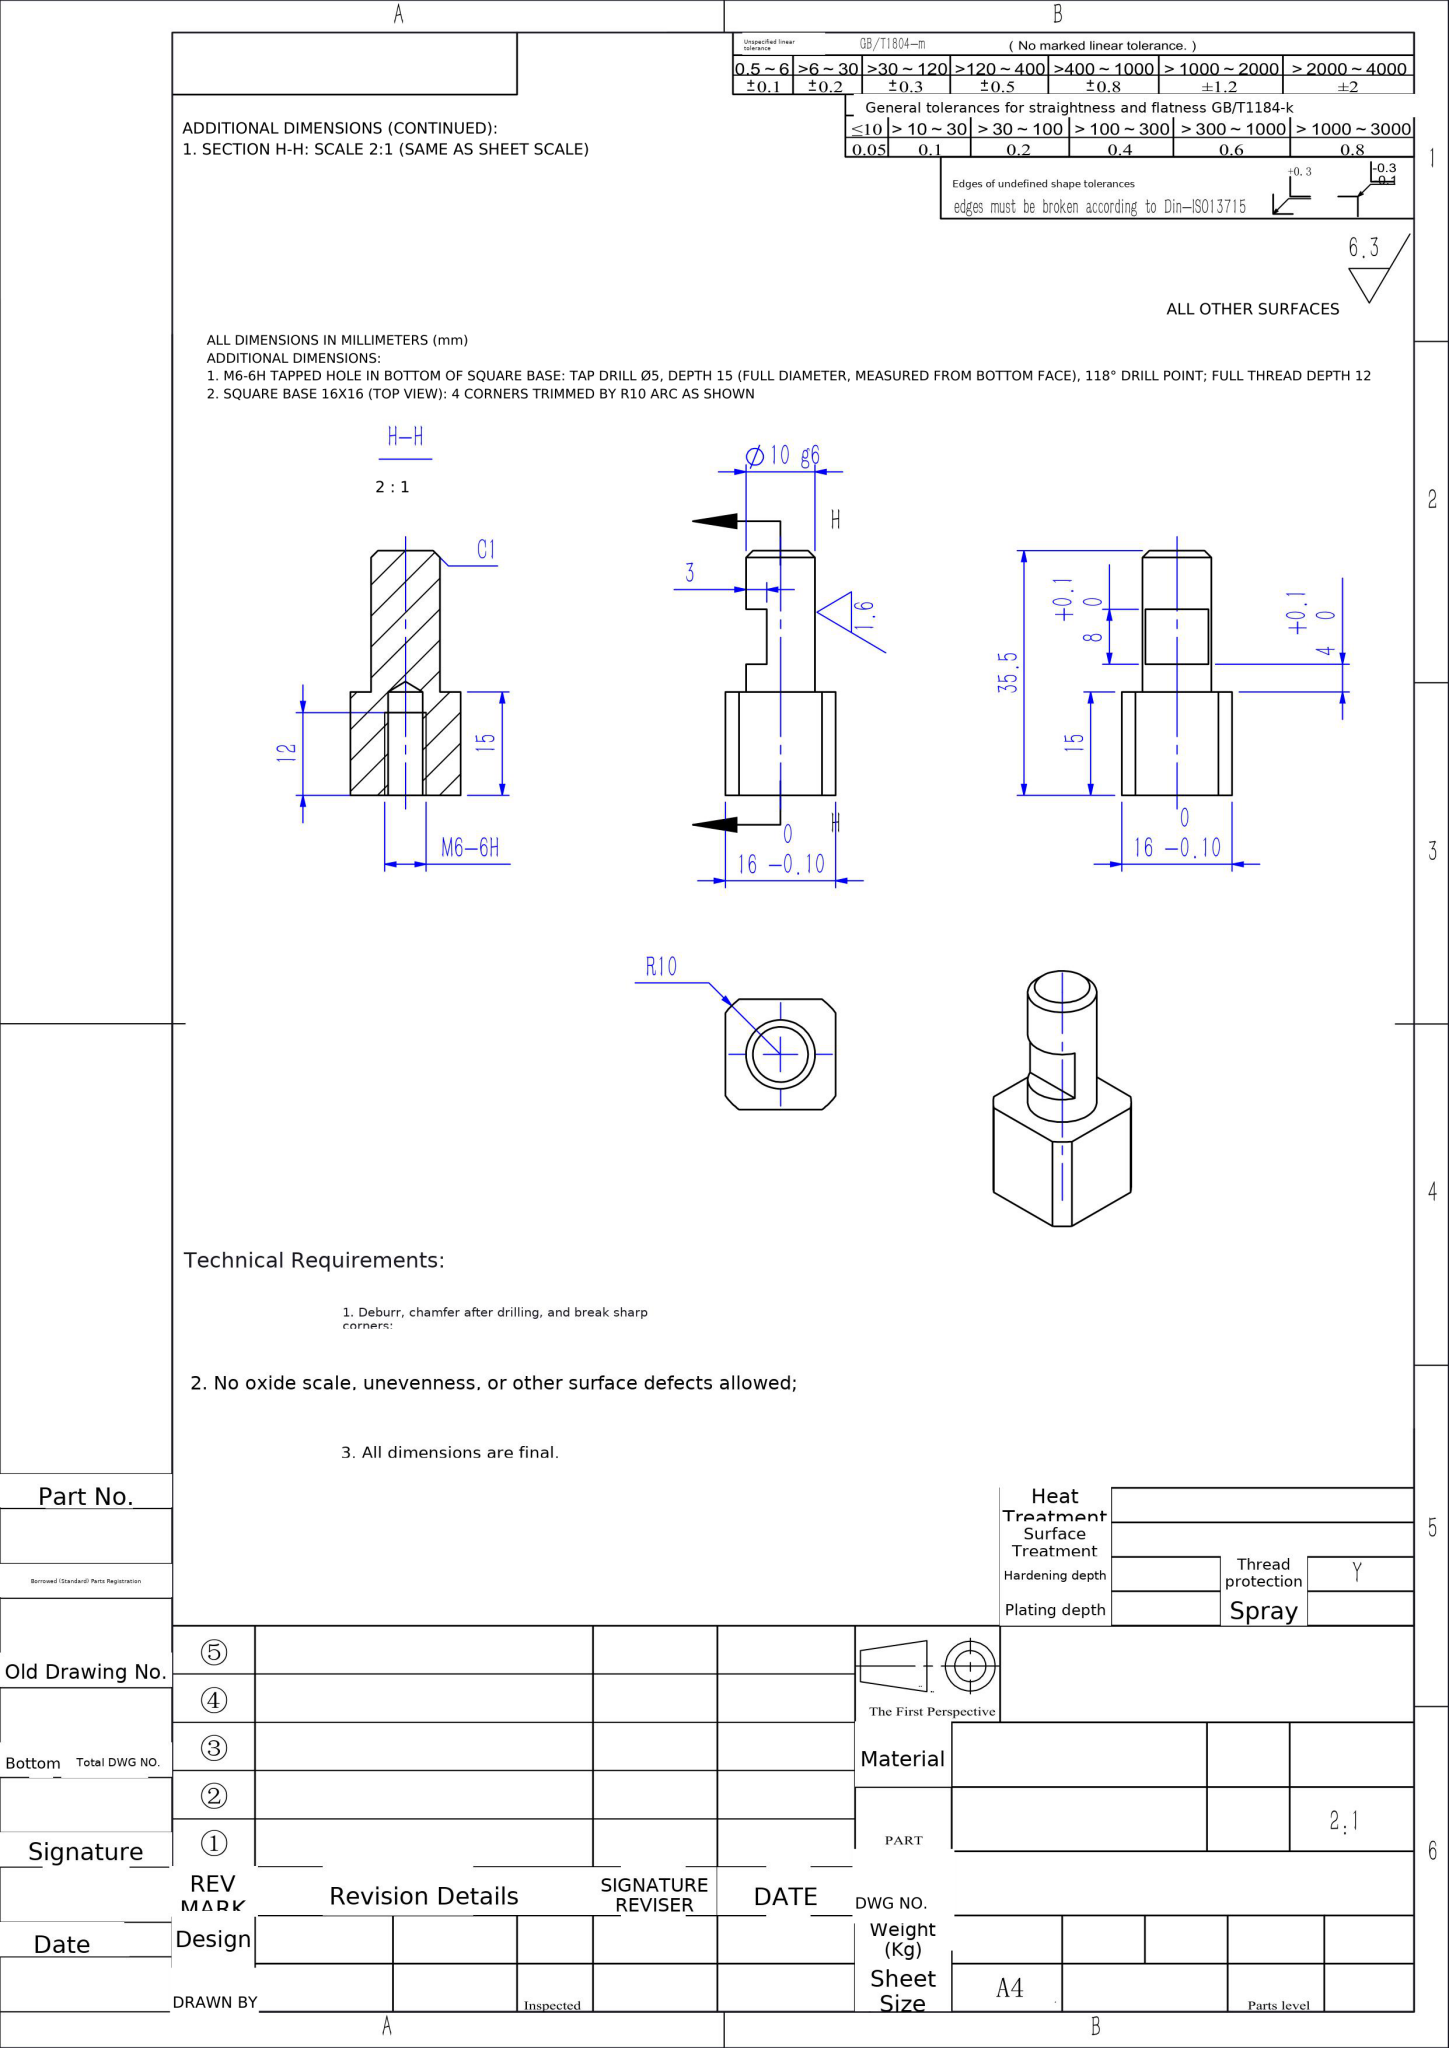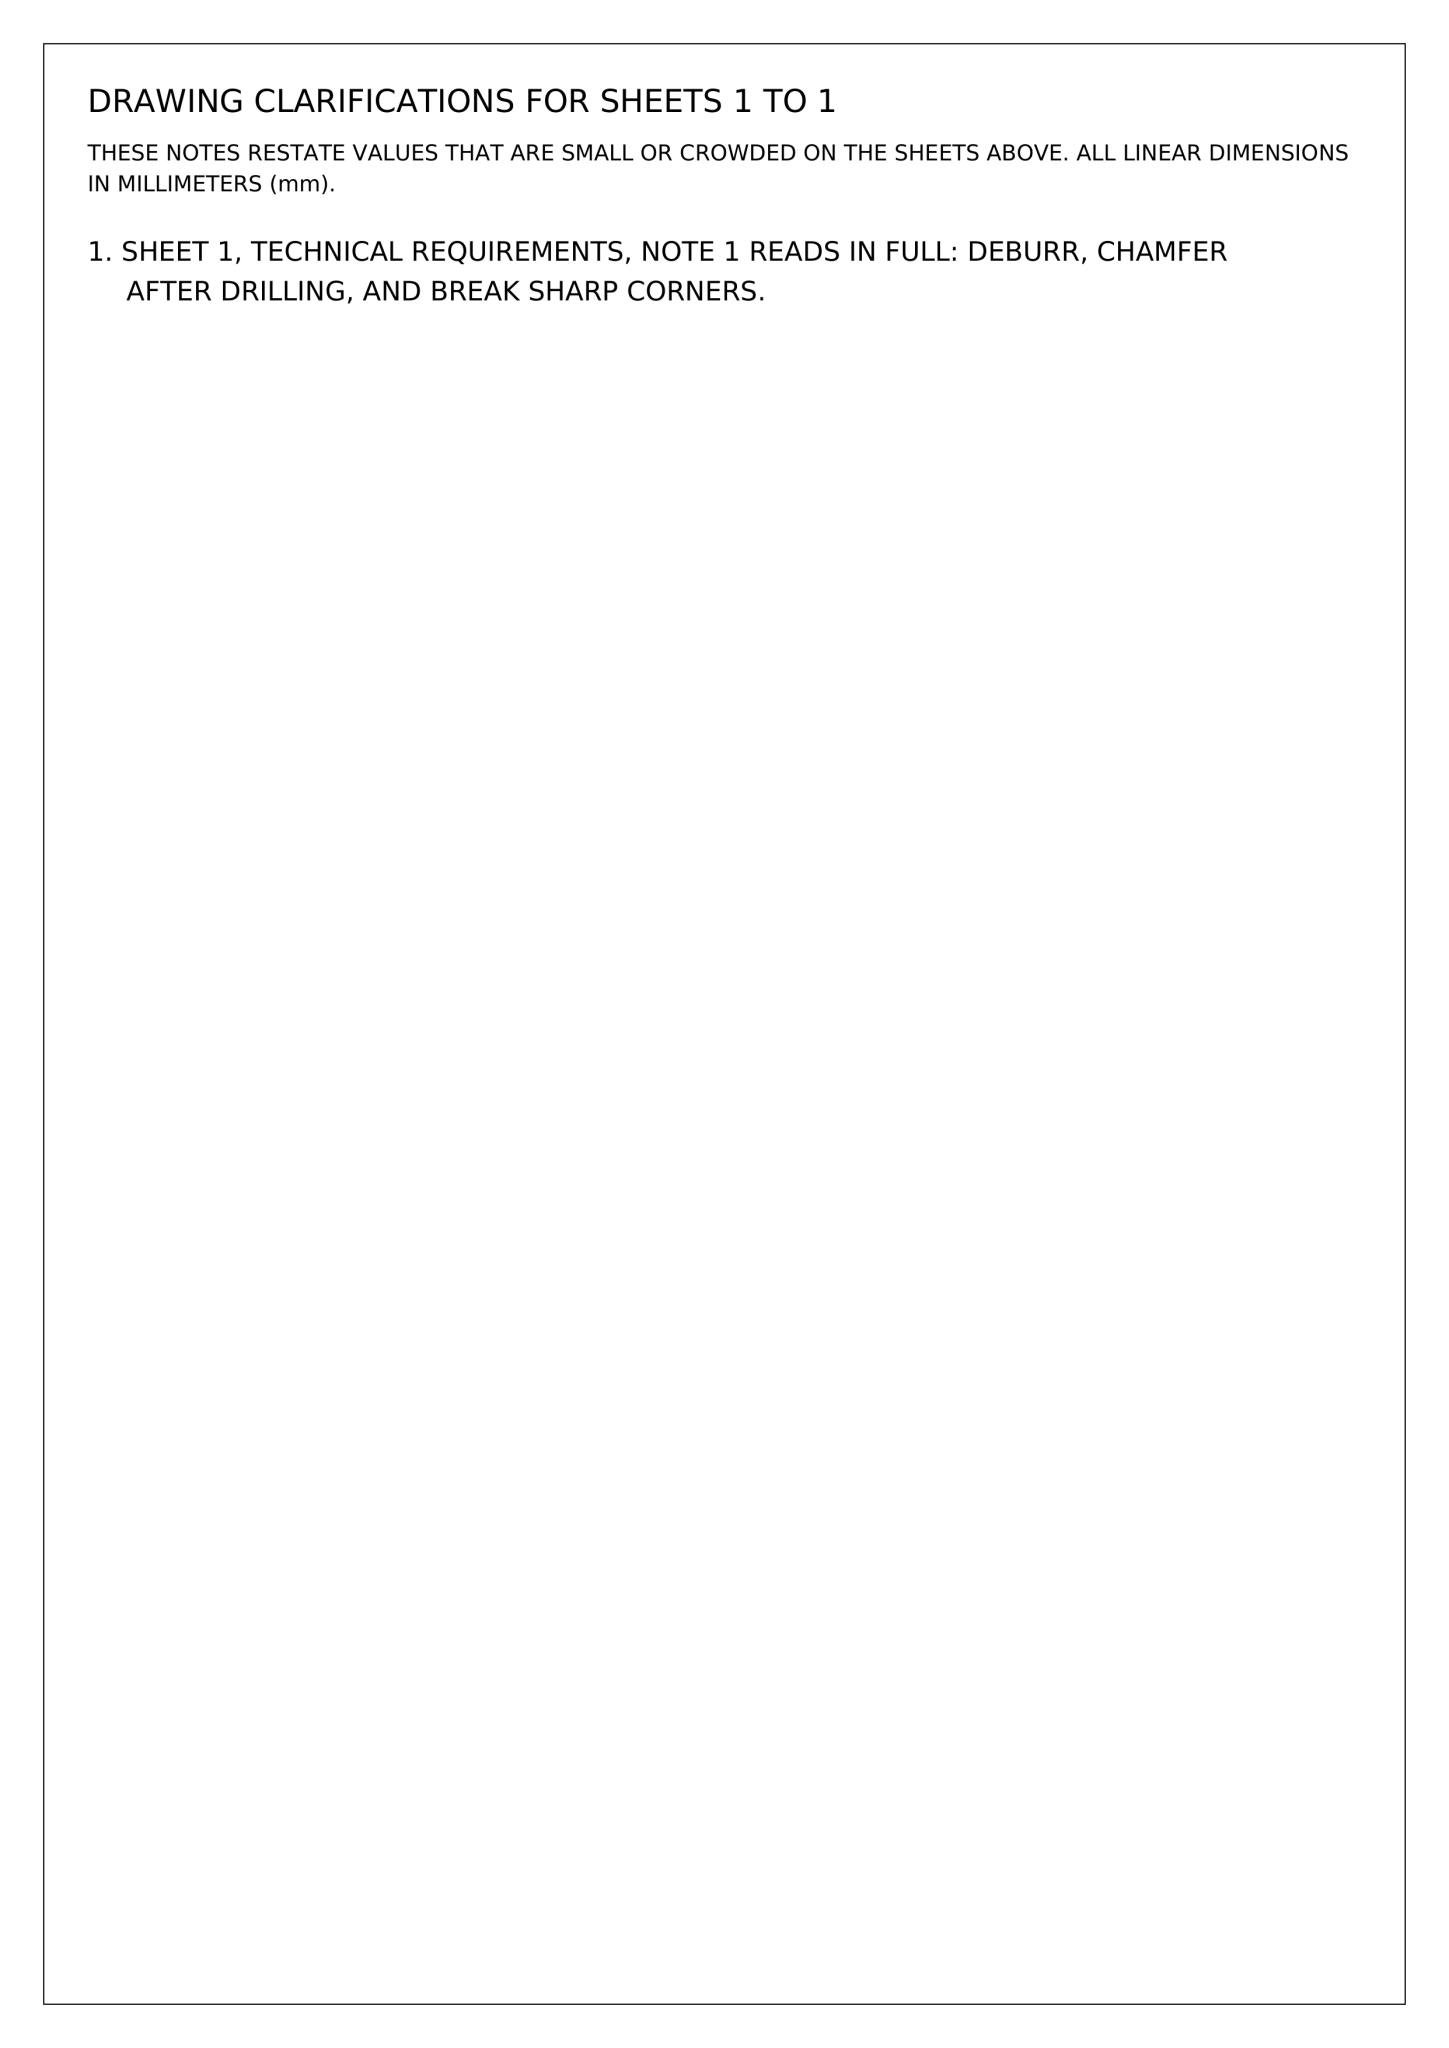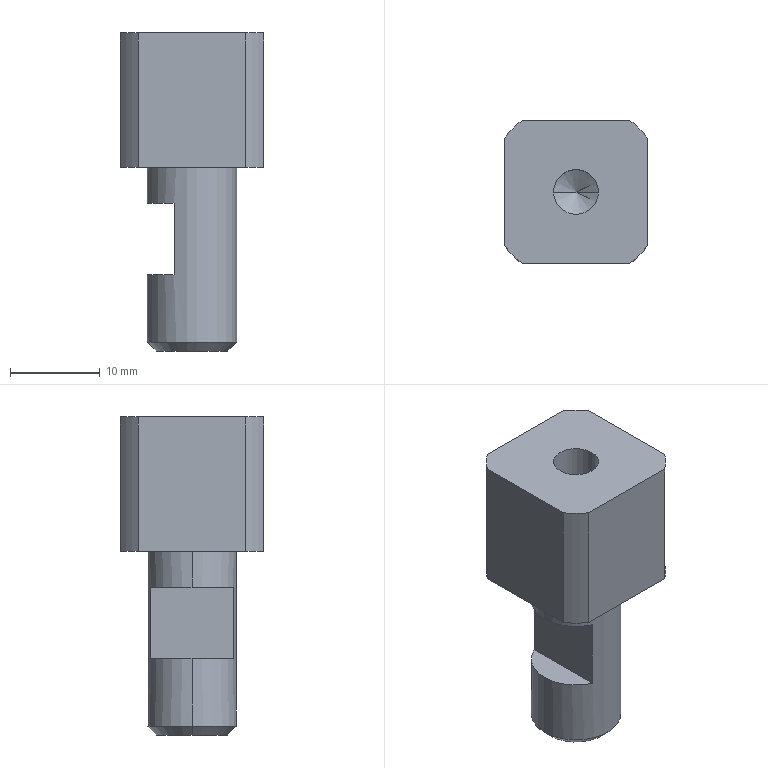Part | NX | mm | 1 solid | 22 faces | box 16 x 16 x 35.5 mm | volume 4864 mm3 | plane 10 | cylinder 8 | cone 4 | commonest cylinder face diameters 20 x4 5 x2 10 x2
STEP:
#1=COLOUR_RGB('',0.6471,0.6196,0.5882);
#2=FILL_AREA_STYLE_COLOUR('',#1);
#3=FILL_AREA_STYLE('',(#2));
#4=SURFACE_STYLE_FILL_AREA(#3);
#5=SURFACE_SIDE_STYLE('',(#4));
#6=SURFACE_STYLE_USAGE(.BOTH.,#5);
#7=PRESENTATION_STYLE_ASSIGNMENT((#6));
#8=CARTESIAN_POINT('',(-2.5,0.,20.5));
#9=VERTEX_POINT('',#8);
#10=CARTESIAN_POINT('',(2.5,0.,20.5));
#11=VERTEX_POINT('',#10);
#12=CARTESIAN_POINT('',(0.,0.,20.5));
#13=DIRECTION('',(0.,0.,1.));
#14=DIRECTION('',(1.,0.,0.));
#15=AXIS2_PLACEMENT_3D('',#12,#13,#14);
#16=CIRCLE('',#15,2.5);
#17=EDGE_CURVE('',#9,#11,#16,.T.);
#18=ORIENTED_EDGE('',*,*,#17,.F.);
#19=CARTESIAN_POINT('',(-2.5,0.,35.5));
#20=VERTEX_POINT('',#19);
#21=CARTESIAN_POINT('',(-2.5,0.,35.5));
#22=DIRECTION('',(0.,0.,1.));
#23=VECTOR('',#22,1000.);
#24=LINE('',#21,#23);
#25=EDGE_CURVE('',#9,#20,#24,.T.);
#26=ORIENTED_EDGE('',*,*,#25,.T.);
#27=CARTESIAN_POINT('',(2.5,0.,35.5));
#28=VERTEX_POINT('',#27);
#29=CARTESIAN_POINT('',(0.,0.,35.5));
#30=DIRECTION('',(0.,0.,1.));
#31=DIRECTION('',(1.,0.,0.));
#32=AXIS2_PLACEMENT_3D('',#29,#30,#31);
#33=CIRCLE('',#32,2.5);
#34=EDGE_CURVE('',#20,#28,#33,.T.);
#35=ORIENTED_EDGE('',*,*,#34,.T.);
#36=CARTESIAN_POINT('',(2.5,0.,35.5));
#37=DIRECTION('',(0.,0.,1.));
#38=VECTOR('',#37,1000.);
#39=LINE('',#36,#38);
#40=EDGE_CURVE('',#11,#28,#39,.T.);
#41=ORIENTED_EDGE('',*,*,#40,.F.);
#42=EDGE_LOOP('',(#18,#26,#35,#41));
#43=FACE_OUTER_BOUND('',#42,.T.);
#44=CARTESIAN_POINT('',(0.,0.,35.5));
#45=DIRECTION('',(0.,0.,1.));
#46=DIRECTION('',(1.,0.,0.));
#47=AXIS2_PLACEMENT_3D('',#44,#45,#46);
#48=CYLINDRICAL_SURFACE('',#47,2.5);
#49=ADVANCED_FACE('',(#43),#48,.F.);
#50=STYLED_ITEM('',(#7),#49);
#51=PRESENTATION_LAYER_ASSIGNMENT('','',(#50));
#52=(LENGTH_UNIT()NAMED_UNIT(*)SI_UNIT(.MILLI.,.METRE.));
#53=UNCERTAINTY_MEASURE_WITH_UNIT(LENGTH_MEASURE(0.00001),#52,'','');
#54=(NAMED_UNIT(*)PLANE_ANGLE_UNIT()SI_UNIT($,.RADIAN.));
#55=(NAMED_UNIT(*)SI_UNIT($,.STERADIAN.)SOLID_ANGLE_UNIT());
#56=(GEOMETRIC_REPRESENTATION_CONTEXT(3)GLOBAL_UNCERTAINTY_ASSIGNED_CONTEXT((#53))GLOBAL_UNIT_ASSIGNED_CONTEXT((#52,#54,#55))REPRESENTATION_CONTEXT('',''));
#57=MECHANICAL_DESIGN_GEOMETRIC_PRESENTATION_REPRESENTATION('',(#50),#56);
#58=COLOUR_RGB('',0.6471,0.6196,0.5882);
#59=FILL_AREA_STYLE_COLOUR('',#58);
#60=FILL_AREA_STYLE('',(#59));
#61=SURFACE_STYLE_FILL_AREA(#60);
#62=SURFACE_SIDE_STYLE('',(#61));
#63=SURFACE_STYLE_USAGE(.BOTH.,#62);
#64=PRESENTATION_STYLE_ASSIGNMENT((#63));
#65=CARTESIAN_POINT('',(-4.,0.,0.));
#66=VERTEX_POINT('',#65);
#67=CARTESIAN_POINT('',(4.,0.,0.));
#68=VERTEX_POINT('',#67);
#69=CARTESIAN_POINT('',(0.,0.,0.));
#70=DIRECTION('',(0.,0.,-1.));
#71=DIRECTION('',(1.,0.,0.));
#72=AXIS2_PLACEMENT_3D('',#69,#70,#71);
#73=CIRCLE('',#72,4.);
#74=EDGE_CURVE('',#66,#68,#73,.T.);
#75=ORIENTED_EDGE('',*,*,#74,.F.);
#76=CARTESIAN_POINT('',(-5.,0.,1.));
#77=VERTEX_POINT('',#76);
#78=CARTESIAN_POINT('',(-5.,0.,1.));
#79=DIRECTION('',(-0.7071,0.,0.7071));
#80=VECTOR('',#79,1000.);
#81=LINE('',#78,#80);
#82=EDGE_CURVE('',#66,#77,#81,.T.);
#83=ORIENTED_EDGE('',*,*,#82,.T.);
#84=CARTESIAN_POINT('',(5.,0.,1.));
#85=VERTEX_POINT('',#84);
#86=CARTESIAN_POINT('',(0.,0.,1.));
#87=DIRECTION('',(0.,0.,1.));
#88=DIRECTION('',(1.,0.,0.));
#89=AXIS2_PLACEMENT_3D('',#86,#87,#88);
#90=CIRCLE('',#89,5.);
#91=EDGE_CURVE('',#85,#77,#90,.T.);
#92=ORIENTED_EDGE('',*,*,#91,.F.);
#93=CARTESIAN_POINT('',(5.,0.,1.));
#94=DIRECTION('',(0.7071,0.,0.7071));
#95=VECTOR('',#94,1000.);
#96=LINE('',#93,#95);
#97=EDGE_CURVE('',#68,#85,#96,.T.);
#98=ORIENTED_EDGE('',*,*,#97,.F.);
#99=EDGE_LOOP('',(#75,#83,#92,#98));
#100=FACE_OUTER_BOUND('',#99,.T.);
#101=CARTESIAN_POINT('',(0.,0.,1.));
#102=DIRECTION('',(0.,0.,1.));
#103=DIRECTION('',(1.,0.,0.));
#104=AXIS2_PLACEMENT_3D('',#101,#102,#103);
#105=CONICAL_SURFACE('',#104,5.,0.7854);
#106=ADVANCED_FACE('',(#100),#105,.T.);
#107=CARTESIAN_POINT('',(-0.,0.,18.998));
#108=VERTEX_POINT('',#107);
#109=CARTESIAN_POINT('',(2.5,0.,20.5));
#110=DIRECTION('',(0.8572,0.,0.515));
#111=VECTOR('',#110,1000.);
#112=LINE('',#109,#111);
#113=EDGE_CURVE('',#108,#11,#112,.T.);
#114=ORIENTED_EDGE('',*,*,#113,.F.);
#115=CARTESIAN_POINT('',(-2.5,0.,20.5));
#116=DIRECTION('',(-0.8572,0.,0.515));
#117=VECTOR('',#116,1000.);
#118=LINE('',#115,#117);
#119=EDGE_CURVE('',#108,#9,#118,.T.);
#120=ORIENTED_EDGE('',*,*,#119,.T.);
#121=ORIENTED_EDGE('',*,*,#17,.T.);
#122=EDGE_LOOP('',(#114,#120,#121));
#123=FACE_OUTER_BOUND('',#122,.T.);
#124=CARTESIAN_POINT('',(0.,0.,20.5));
#125=DIRECTION('',(0.,0.,1.));
#126=DIRECTION('',(1.,0.,0.));
#127=AXIS2_PLACEMENT_3D('',#124,#125,#126);
#128=CONICAL_SURFACE('',#127,2.5,1.03);
#129=ADVANCED_FACE('',(#123),#128,.F.);
#130=CARTESIAN_POINT('',(5.,0.,20.5));
#131=VERTEX_POINT('',#130);
#132=CARTESIAN_POINT('',(-5.,0.,20.5));
#133=VERTEX_POINT('',#132);
#134=CARTESIAN_POINT('',(0.,0.,20.5));
#135=DIRECTION('',(0.,0.,1.));
#136=DIRECTION('',(1.,0.,0.));
#137=AXIS2_PLACEMENT_3D('',#134,#135,#136);
#138=CIRCLE('',#137,5.);
#139=EDGE_CURVE('',#131,#133,#138,.T.);
#140=ORIENTED_EDGE('',*,*,#139,.F.);
#141=CARTESIAN_POINT('',(5.,0.,35.5));
#142=DIRECTION('',(0.,0.,-1.));
#143=VECTOR('',#142,1000.);
#144=LINE('',#141,#143);
#145=EDGE_CURVE('',#131,#85,#144,.T.);
#146=ORIENTED_EDGE('',*,*,#145,.T.);
#147=ORIENTED_EDGE('',*,*,#91,.T.);
#148=CARTESIAN_POINT('',(-5.,0.,8.5));
#149=VERTEX_POINT('',#148);
#150=CARTESIAN_POINT('',(-5.,0.,35.5));
#151=DIRECTION('',(0.,0.,-1.));
#152=VECTOR('',#151,1000.);
#153=LINE('',#150,#152);
#154=EDGE_CURVE('',#149,#77,#153,.T.);
#155=ORIENTED_EDGE('',*,*,#154,.F.);
#156=CARTESIAN_POINT('',(-2.,4.583,8.5));
#157=VERTEX_POINT('',#156);
#158=CARTESIAN_POINT('',(0.,0.,8.5));
#159=DIRECTION('',(0.,0.,-1.));
#160=DIRECTION('',(-1.,0.,0.));
#161=AXIS2_PLACEMENT_3D('',#158,#159,#160);
#162=CIRCLE('',#161,5.);
#163=EDGE_CURVE('',#149,#157,#162,.T.);
#164=ORIENTED_EDGE('',*,*,#163,.T.);
#165=CARTESIAN_POINT('',(-2.,4.583,16.5));
#166=VERTEX_POINT('',#165);
#167=CARTESIAN_POINT('',(-2.,4.583,35.5));
#168=DIRECTION('',(0.,0.,1.));
#169=VECTOR('',#168,1000.);
#170=LINE('',#167,#169);
#171=EDGE_CURVE('',#157,#166,#170,.T.);
#172=ORIENTED_EDGE('',*,*,#171,.T.);
#173=CARTESIAN_POINT('',(-5.,0.,16.5));
#174=VERTEX_POINT('',#173);
#175=CARTESIAN_POINT('',(0.,0.,16.5));
#176=DIRECTION('',(0.,0.,-1.));
#177=DIRECTION('',(-1.,0.,0.));
#178=AXIS2_PLACEMENT_3D('',#175,#176,#177);
#179=CIRCLE('',#178,5.);
#180=EDGE_CURVE('',#174,#166,#179,.T.);
#181=ORIENTED_EDGE('',*,*,#180,.F.);
#182=CARTESIAN_POINT('',(-5.,0.,35.5));
#183=DIRECTION('',(0.,0.,-1.));
#184=VECTOR('',#183,1000.);
#185=LINE('',#182,#184);
#186=EDGE_CURVE('',#133,#174,#185,.T.);
#187=ORIENTED_EDGE('',*,*,#186,.F.);
#188=EDGE_LOOP('',(#140,#146,#147,#155,#164,#172,#181,#187));
#189=FACE_OUTER_BOUND('',#188,.T.);
#190=CARTESIAN_POINT('',(0.,0.,35.5));
#191=DIRECTION('',(0.,0.,-1.));
#192=DIRECTION('',(-1.,0.,0.));
#193=AXIS2_PLACEMENT_3D('',#190,#191,#192);
#194=CYLINDRICAL_SURFACE('',#193,5.);
#195=ADVANCED_FACE('',(#189),#194,.T.);
#196=CARTESIAN_POINT('',(-8.,-6.,35.5));
#197=VERTEX_POINT('',#196);
#198=CARTESIAN_POINT('',(-6.,-8.,35.5));
#199=VERTEX_POINT('',#198);
#200=CARTESIAN_POINT('',(0.,0.,35.5));
#201=DIRECTION('',(0.,0.,1.));
#202=DIRECTION('',(1.,0.,0.));
#203=AXIS2_PLACEMENT_3D('',#200,#201,#202);
#204=CIRCLE('',#203,10.);
#205=EDGE_CURVE('',#197,#199,#204,.T.);
#206=ORIENTED_EDGE('',*,*,#205,.F.);
#207=CARTESIAN_POINT('',(-8.,-6.,20.5));
#208=VERTEX_POINT('',#207);
#209=CARTESIAN_POINT('',(-8.,-6.,20.5));
#210=DIRECTION('',(0.,0.,-1.));
#211=VECTOR('',#210,1000.);
#212=LINE('',#209,#211);
#213=EDGE_CURVE('',#197,#208,#212,.T.);
#214=ORIENTED_EDGE('',*,*,#213,.T.);
#215=CARTESIAN_POINT('',(-6.,-8.,20.5));
#216=VERTEX_POINT('',#215);
#217=CARTESIAN_POINT('',(0.,0.,20.5));
#218=DIRECTION('',(0.,0.,1.));
#219=DIRECTION('',(1.,0.,0.));
#220=AXIS2_PLACEMENT_3D('',#217,#218,#219);
#221=CIRCLE('',#220,10.);
#222=EDGE_CURVE('',#208,#216,#221,.T.);
#223=ORIENTED_EDGE('',*,*,#222,.T.);
#224=CARTESIAN_POINT('',(-6.,-8.,20.5));
#225=DIRECTION('',(0.,0.,1.));
#226=VECTOR('',#225,1000.);
#227=LINE('',#224,#226);
#228=EDGE_CURVE('',#216,#199,#227,.T.);
#229=ORIENTED_EDGE('',*,*,#228,.T.);
#230=EDGE_LOOP('',(#206,#214,#223,#229));
#231=FACE_OUTER_BOUND('',#230,.T.);
#232=CARTESIAN_POINT('',(0.,0.,20.5));
#233=DIRECTION('',(0.,0.,1.));
#234=DIRECTION('',(1.,0.,0.));
#235=AXIS2_PLACEMENT_3D('',#232,#233,#234);
#236=CYLINDRICAL_SURFACE('',#235,10.);
#237=ADVANCED_FACE('',(#231),#236,.T.);
#238=CARTESIAN_POINT('',(-6.,8.,20.5));
#239=VERTEX_POINT('',#238);
#240=CARTESIAN_POINT('',(-8.,6.,20.5));
#241=VERTEX_POINT('',#240);
#242=CARTESIAN_POINT('',(0.,0.,20.5));
#243=DIRECTION('',(0.,0.,1.));
#244=DIRECTION('',(1.,0.,0.));
#245=AXIS2_PLACEMENT_3D('',#242,#243,#244);
#246=CIRCLE('',#245,10.);
#247=EDGE_CURVE('',#239,#241,#246,.T.);
#248=ORIENTED_EDGE('',*,*,#247,.T.);
#249=CARTESIAN_POINT('',(-8.,6.,35.5));
#250=VERTEX_POINT('',#249);
#251=CARTESIAN_POINT('',(-8.,6.,20.5));
#252=DIRECTION('',(0.,0.,1.));
#253=VECTOR('',#252,1000.);
#254=LINE('',#251,#253);
#255=EDGE_CURVE('',#241,#250,#254,.T.);
#256=ORIENTED_EDGE('',*,*,#255,.T.);
#257=CARTESIAN_POINT('',(-6.,8.,35.5));
#258=VERTEX_POINT('',#257);
#259=CARTESIAN_POINT('',(0.,0.,35.5));
#260=DIRECTION('',(0.,0.,1.));
#261=DIRECTION('',(1.,0.,0.));
#262=AXIS2_PLACEMENT_3D('',#259,#260,#261);
#263=CIRCLE('',#262,10.);
#264=EDGE_CURVE('',#258,#250,#263,.T.);
#265=ORIENTED_EDGE('',*,*,#264,.F.);
#266=CARTESIAN_POINT('',(-6.,8.,20.5));
#267=DIRECTION('',(0.,0.,-1.));
#268=VECTOR('',#267,1000.);
#269=LINE('',#266,#268);
#270=EDGE_CURVE('',#258,#239,#269,.T.);
#271=ORIENTED_EDGE('',*,*,#270,.T.);
#272=EDGE_LOOP('',(#248,#256,#265,#271));
#273=FACE_OUTER_BOUND('',#272,.T.);
#274=CARTESIAN_POINT('',(0.,0.,20.5));
#275=DIRECTION('',(0.,0.,1.));
#276=DIRECTION('',(1.,0.,0.));
#277=AXIS2_PLACEMENT_3D('',#274,#275,#276);
#278=CYLINDRICAL_SURFACE('',#277,10.);
#279=ADVANCED_FACE('',(#273),#278,.T.);
#280=CARTESIAN_POINT('',(8.,6.,20.5));
#281=VERTEX_POINT('',#280);
#282=CARTESIAN_POINT('',(6.,8.,20.5));
#283=VERTEX_POINT('',#282);
#284=CARTESIAN_POINT('',(0.,0.,20.5));
#285=DIRECTION('',(0.,0.,1.));
#286=DIRECTION('',(1.,0.,0.));
#287=AXIS2_PLACEMENT_3D('',#284,#285,#286);
#288=CIRCLE('',#287,10.);
#289=EDGE_CURVE('',#281,#283,#288,.T.);
#290=ORIENTED_EDGE('',*,*,#289,.T.);
#291=CARTESIAN_POINT('',(6.,8.,35.5));
#292=VERTEX_POINT('',#291);
#293=CARTESIAN_POINT('',(6.,8.,20.5));
#294=DIRECTION('',(0.,0.,1.));
#295=VECTOR('',#294,1000.);
#296=LINE('',#293,#295);
#297=EDGE_CURVE('',#283,#292,#296,.T.);
#298=ORIENTED_EDGE('',*,*,#297,.T.);
#299=CARTESIAN_POINT('',(8.,6.,35.5));
#300=VERTEX_POINT('',#299);
#301=CARTESIAN_POINT('',(0.,0.,35.5));
#302=DIRECTION('',(0.,0.,1.));
#303=DIRECTION('',(1.,0.,0.));
#304=AXIS2_PLACEMENT_3D('',#301,#302,#303);
#305=CIRCLE('',#304,10.);
#306=EDGE_CURVE('',#300,#292,#305,.T.);
#307=ORIENTED_EDGE('',*,*,#306,.F.);
#308=CARTESIAN_POINT('',(8.,6.,20.5));
#309=DIRECTION('',(0.,0.,-1.));
#310=VECTOR('',#309,1000.);
#311=LINE('',#308,#310);
#312=EDGE_CURVE('',#300,#281,#311,.T.);
#313=ORIENTED_EDGE('',*,*,#312,.T.);
#314=EDGE_LOOP('',(#290,#298,#307,#313));
#315=FACE_OUTER_BOUND('',#314,.T.);
#316=CARTESIAN_POINT('',(0.,0.,20.5));
#317=DIRECTION('',(0.,0.,1.));
#318=DIRECTION('',(1.,0.,0.));
#319=AXIS2_PLACEMENT_3D('',#316,#317,#318);
#320=CYLINDRICAL_SURFACE('',#319,10.);
#321=ADVANCED_FACE('',(#315),#320,.T.);
#322=CARTESIAN_POINT('',(6.,-8.,20.5));
#323=VERTEX_POINT('',#322);
#324=CARTESIAN_POINT('',(8.,-6.,20.5));
#325=VERTEX_POINT('',#324);
#326=CARTESIAN_POINT('',(0.,0.,20.5));
#327=DIRECTION('',(0.,0.,1.));
#328=DIRECTION('',(1.,0.,0.));
#329=AXIS2_PLACEMENT_3D('',#326,#327,#328);
#330=CIRCLE('',#329,10.);
#331=EDGE_CURVE('',#323,#325,#330,.T.);
#332=ORIENTED_EDGE('',*,*,#331,.T.);
#333=CARTESIAN_POINT('',(8.,-6.,35.5));
#334=VERTEX_POINT('',#333);
#335=CARTESIAN_POINT('',(8.,-6.,20.5));
#336=DIRECTION('',(0.,0.,1.));
#337=VECTOR('',#336,1000.);
#338=LINE('',#335,#337);
#339=EDGE_CURVE('',#325,#334,#338,.T.);
#340=ORIENTED_EDGE('',*,*,#339,.T.);
#341=CARTESIAN_POINT('',(6.,-8.,35.5));
#342=VERTEX_POINT('',#341);
#343=CARTESIAN_POINT('',(0.,0.,35.5));
#344=DIRECTION('',(0.,0.,1.));
#345=DIRECTION('',(1.,0.,0.));
#346=AXIS2_PLACEMENT_3D('',#343,#344,#345);
#347=CIRCLE('',#346,10.);
#348=EDGE_CURVE('',#342,#334,#347,.T.);
#349=ORIENTED_EDGE('',*,*,#348,.F.);
#350=CARTESIAN_POINT('',(6.,-8.,20.5));
#351=DIRECTION('',(0.,0.,-1.));
#352=VECTOR('',#351,1000.);
#353=LINE('',#350,#352);
#354=EDGE_CURVE('',#342,#323,#353,.T.);
#355=ORIENTED_EDGE('',*,*,#354,.T.);
#356=EDGE_LOOP('',(#332,#340,#349,#355));
#357=FACE_OUTER_BOUND('',#356,.T.);
#358=CARTESIAN_POINT('',(0.,0.,20.5));
#359=DIRECTION('',(0.,0.,1.));
#360=DIRECTION('',(1.,0.,0.));
#361=AXIS2_PLACEMENT_3D('',#358,#359,#360);
#362=CYLINDRICAL_SURFACE('',#361,10.);
#363=ADVANCED_FACE('',(#357),#362,.T.);
#364=CARTESIAN_POINT('',(0.,0.,20.5));
#365=DIRECTION('',(0.,0.,1.));
#366=DIRECTION('',(1.,0.,0.));
#367=AXIS2_PLACEMENT_3D('',#364,#365,#366);
#368=CIRCLE('',#367,5.);
#369=EDGE_CURVE('',#133,#131,#368,.T.);
#370=ORIENTED_EDGE('',*,*,#369,.T.);
#371=ORIENTED_EDGE('',*,*,#139,.T.);
#372=EDGE_LOOP('',(#370,#371));
#373=FACE_BOUND('',#372,.T.);
#374=CARTESIAN_POINT('',(-8.,8.,20.5));
#375=DIRECTION('',(0.,-1.,0.));
#376=VECTOR('',#375,1000.);
#377=LINE('',#374,#376);
#378=EDGE_CURVE('',#241,#208,#377,.T.);
#379=ORIENTED_EDGE('',*,*,#378,.F.);
#380=ORIENTED_EDGE('',*,*,#247,.F.);
#381=CARTESIAN_POINT('',(-8.,8.,20.5));
#382=DIRECTION('',(-1.,0.,0.));
#383=VECTOR('',#382,1000.);
#384=LINE('',#381,#383);
#385=EDGE_CURVE('',#283,#239,#384,.T.);
#386=ORIENTED_EDGE('',*,*,#385,.F.);
#387=ORIENTED_EDGE('',*,*,#289,.F.);
#388=CARTESIAN_POINT('',(8.,8.,20.5));
#389=DIRECTION('',(0.,1.,0.));
#390=VECTOR('',#389,1000.);
#391=LINE('',#388,#390);
#392=EDGE_CURVE('',#325,#281,#391,.T.);
#393=ORIENTED_EDGE('',*,*,#392,.F.);
#394=ORIENTED_EDGE('',*,*,#331,.F.);
#395=CARTESIAN_POINT('',(-8.,-8.,20.5));
#396=DIRECTION('',(1.,0.,0.));
#397=VECTOR('',#396,1000.);
#398=LINE('',#395,#397);
#399=EDGE_CURVE('',#216,#323,#398,.T.);
#400=ORIENTED_EDGE('',*,*,#399,.F.);
#401=ORIENTED_EDGE('',*,*,#222,.F.);
#402=EDGE_LOOP('',(#379,#380,#386,#387,#393,#394,#400,#401));
#403=FACE_OUTER_BOUND('',#402,.T.);
#404=CARTESIAN_POINT('',(0.,0.,20.5));
#405=DIRECTION('',(0.,0.,1.));
#406=DIRECTION('',(1.,0.,0.));
#407=AXIS2_PLACEMENT_3D('',#404,#405,#406);
#408=PLANE('',#407);
#409=ADVANCED_FACE('',(#373,#403),#408,.F.);
#410=CARTESIAN_POINT('',(0.,0.,35.5));
#411=DIRECTION('',(0.,0.,1.));
#412=DIRECTION('',(1.,0.,0.));
#413=AXIS2_PLACEMENT_3D('',#410,#411,#412);
#414=CIRCLE('',#413,2.5);
#415=EDGE_CURVE('',#28,#20,#414,.T.);
#416=ORIENTED_EDGE('',*,*,#415,.F.);
#417=ORIENTED_EDGE('',*,*,#34,.F.);
#418=EDGE_LOOP('',(#416,#417));
#419=FACE_BOUND('',#418,.T.);
#420=ORIENTED_EDGE('',*,*,#264,.T.);
#421=CARTESIAN_POINT('',(-8.,0.,35.5));
#422=DIRECTION('',(0.,-1.,0.));
#423=VECTOR('',#422,1000.);
#424=LINE('',#421,#423);
#425=EDGE_CURVE('',#250,#197,#424,.T.);
#426=ORIENTED_EDGE('',*,*,#425,.T.);
#427=ORIENTED_EDGE('',*,*,#205,.T.);
#428=CARTESIAN_POINT('',(0.,-8.,35.5));
#429=DIRECTION('',(1.,0.,0.));
#430=VECTOR('',#429,1000.);
#431=LINE('',#428,#430);
#432=EDGE_CURVE('',#199,#342,#431,.T.);
#433=ORIENTED_EDGE('',*,*,#432,.T.);
#434=ORIENTED_EDGE('',*,*,#348,.T.);
#435=CARTESIAN_POINT('',(8.,0.,35.5));
#436=DIRECTION('',(0.,1.,0.));
#437=VECTOR('',#436,1000.);
#438=LINE('',#435,#437);
#439=EDGE_CURVE('',#334,#300,#438,.T.);
#440=ORIENTED_EDGE('',*,*,#439,.T.);
#441=ORIENTED_EDGE('',*,*,#306,.T.);
#442=CARTESIAN_POINT('',(0.,8.,35.5));
#443=DIRECTION('',(-1.,0.,0.));
#444=VECTOR('',#443,1000.);
#445=LINE('',#442,#444);
#446=EDGE_CURVE('',#292,#258,#445,.T.);
#447=ORIENTED_EDGE('',*,*,#446,.T.);
#448=EDGE_LOOP('',(#420,#426,#427,#433,#434,#440,#441,#447));
#449=FACE_OUTER_BOUND('',#448,.T.);
#450=CARTESIAN_POINT('',(0.,0.,35.5));
#451=DIRECTION('',(0.,0.,1.));
#452=DIRECTION('',(1.,0.,0.));
#453=AXIS2_PLACEMENT_3D('',#450,#451,#452);
#454=PLANE('',#453);
#455=ADVANCED_FACE('',(#419,#449),#454,.T.);
#456=ORIENTED_EDGE('',*,*,#145,.F.);
#457=ORIENTED_EDGE('',*,*,#369,.F.);
#458=ORIENTED_EDGE('',*,*,#186,.T.);
#459=CARTESIAN_POINT('',(-2.,-4.583,16.5));
#460=VERTEX_POINT('',#459);
#461=CARTESIAN_POINT('',(0.,0.,16.5));
#462=DIRECTION('',(0.,0.,-1.));
#463=DIRECTION('',(-1.,0.,0.));
#464=AXIS2_PLACEMENT_3D('',#461,#462,#463);
#465=CIRCLE('',#464,5.);
#466=EDGE_CURVE('',#460,#174,#465,.T.);
#467=ORIENTED_EDGE('',*,*,#466,.F.);
#468=CARTESIAN_POINT('',(-2.,-4.583,8.5));
#469=VERTEX_POINT('',#468);
#470=CARTESIAN_POINT('',(-2.,-4.583,35.5));
#471=DIRECTION('',(0.,0.,-1.));
#472=VECTOR('',#471,1000.);
#473=LINE('',#470,#472);
#474=EDGE_CURVE('',#460,#469,#473,.T.);
#475=ORIENTED_EDGE('',*,*,#474,.T.);
#476=CARTESIAN_POINT('',(0.,0.,8.5));
#477=DIRECTION('',(0.,0.,-1.));
#478=DIRECTION('',(-1.,0.,0.));
#479=AXIS2_PLACEMENT_3D('',#476,#477,#478);
#480=CIRCLE('',#479,5.);
#481=EDGE_CURVE('',#469,#149,#480,.T.);
#482=ORIENTED_EDGE('',*,*,#481,.T.);
#483=ORIENTED_EDGE('',*,*,#154,.T.);
#484=CARTESIAN_POINT('',(0.,0.,1.));
#485=DIRECTION('',(0.,0.,1.));
#486=DIRECTION('',(1.,0.,0.));
#487=AXIS2_PLACEMENT_3D('',#484,#485,#486);
#488=CIRCLE('',#487,5.);
#489=EDGE_CURVE('',#77,#85,#488,.T.);
#490=ORIENTED_EDGE('',*,*,#489,.T.);
#491=EDGE_LOOP('',(#456,#457,#458,#467,#475,#482,#483,#490));
#492=FACE_OUTER_BOUND('',#491,.T.);
#493=CARTESIAN_POINT('',(0.,0.,35.5));
#494=DIRECTION('',(0.,0.,-1.));
#495=DIRECTION('',(-1.,0.,0.));
#496=AXIS2_PLACEMENT_3D('',#493,#494,#495);
#497=CYLINDRICAL_SURFACE('',#496,5.);
#498=ADVANCED_FACE('',(#492),#497,.T.);
#499=CARTESIAN_POINT('',(0.,0.,0.));
#500=DIRECTION('',(0.,0.,-1.));
#501=DIRECTION('',(1.,0.,0.));
#502=AXIS2_PLACEMENT_3D('',#499,#500,#501);
#503=CIRCLE('',#502,4.);
#504=EDGE_CURVE('',#68,#66,#503,.T.);
#505=ORIENTED_EDGE('',*,*,#504,.T.);
#506=ORIENTED_EDGE('',*,*,#74,.T.);
#507=EDGE_LOOP('',(#505,#506));
#508=FACE_OUTER_BOUND('',#507,.T.);
#509=CARTESIAN_POINT('',(0.,0.,0.));
#510=DIRECTION('',(0.,0.,1.));
#511=DIRECTION('',(1.,0.,0.));
#512=AXIS2_PLACEMENT_3D('',#509,#510,#511);
#513=PLANE('',#512);
#514=ADVANCED_FACE('',(#508),#513,.F.);
#515=CARTESIAN_POINT('',(-2.,5.,16.5));
#516=DIRECTION('',(0.,-1.,0.));
#517=VECTOR('',#516,1000.);
#518=LINE('',#515,#517);
#519=EDGE_CURVE('',#166,#460,#518,.T.);
#520=ORIENTED_EDGE('',*,*,#519,.F.);
#521=ORIENTED_EDGE('',*,*,#171,.F.);
#522=CARTESIAN_POINT('',(-2.,5.,8.5));
#523=DIRECTION('',(0.,-1.,0.));
#524=VECTOR('',#523,1000.);
#525=LINE('',#522,#524);
#526=EDGE_CURVE('',#157,#469,#525,.T.);
#527=ORIENTED_EDGE('',*,*,#526,.T.);
#528=ORIENTED_EDGE('',*,*,#474,.F.);
#529=EDGE_LOOP('',(#520,#521,#527,#528));
#530=FACE_OUTER_BOUND('',#529,.T.);
#531=CARTESIAN_POINT('',(-2.,5.,16.5));
#532=DIRECTION('',(1.,0.,0.));
#533=DIRECTION('',(0.,0.,-1.));
#534=AXIS2_PLACEMENT_3D('',#531,#532,#533);
#535=PLANE('',#534);
#536=ADVANCED_FACE('',(#530),#535,.F.);
#537=ORIENTED_EDGE('',*,*,#466,.T.);
#538=ORIENTED_EDGE('',*,*,#180,.T.);
#539=ORIENTED_EDGE('',*,*,#519,.T.);
#540=EDGE_LOOP('',(#537,#538,#539));
#541=FACE_OUTER_BOUND('',#540,.T.);
#542=CARTESIAN_POINT('',(0.,0.,16.5));
#543=DIRECTION('',(0.,0.,-1.));
#544=DIRECTION('',(-1.,0.,0.));
#545=AXIS2_PLACEMENT_3D('',#542,#543,#544);
#546=PLANE('',#545);
#547=ADVANCED_FACE('',(#541),#546,.T.);
#548=ORIENTED_EDGE('',*,*,#481,.F.);
#549=ORIENTED_EDGE('',*,*,#526,.F.);
#550=ORIENTED_EDGE('',*,*,#163,.F.);
#551=EDGE_LOOP('',(#548,#549,#550));
#552=FACE_OUTER_BOUND('',#551,.T.);
#553=CARTESIAN_POINT('',(0.,0.,8.5));
#554=DIRECTION('',(0.,0.,-1.));
#555=DIRECTION('',(-1.,0.,0.));
#556=AXIS2_PLACEMENT_3D('',#553,#554,#555);
#557=PLANE('',#556);
#558=ADVANCED_FACE('',(#552),#557,.F.);
#559=ORIENTED_EDGE('',*,*,#432,.F.);
#560=ORIENTED_EDGE('',*,*,#228,.F.);
#561=ORIENTED_EDGE('',*,*,#399,.T.);
#562=ORIENTED_EDGE('',*,*,#354,.F.);
#563=EDGE_LOOP('',(#559,#560,#561,#562));
#564=FACE_OUTER_BOUND('',#563,.T.);
#565=CARTESIAN_POINT('',(-8.,-8.,20.5));
#566=DIRECTION('',(0.,-1.,0.));
#567=DIRECTION('',(0.,0.,-1.));
#568=AXIS2_PLACEMENT_3D('',#565,#566,#567);
#569=PLANE('',#568);
#570=ADVANCED_FACE('',(#564),#569,.T.);
#571=ORIENTED_EDGE('',*,*,#439,.F.);
#572=ORIENTED_EDGE('',*,*,#339,.F.);
#573=ORIENTED_EDGE('',*,*,#392,.T.);
#574=ORIENTED_EDGE('',*,*,#312,.F.);
#575=EDGE_LOOP('',(#571,#572,#573,#574));
#576=FACE_OUTER_BOUND('',#575,.T.);
#577=CARTESIAN_POINT('',(8.,8.,20.5));
#578=DIRECTION('',(1.,0.,0.));
#579=DIRECTION('',(0.,0.,-1.));
#580=AXIS2_PLACEMENT_3D('',#577,#578,#579);
#581=PLANE('',#580);
#582=ADVANCED_FACE('',(#576),#581,.T.);
#583=ORIENTED_EDGE('',*,*,#446,.F.);
#584=ORIENTED_EDGE('',*,*,#297,.F.);
#585=ORIENTED_EDGE('',*,*,#385,.T.);
#586=ORIENTED_EDGE('',*,*,#270,.F.);
#587=EDGE_LOOP('',(#583,#584,#585,#586));
#588=FACE_OUTER_BOUND('',#587,.T.);
#589=CARTESIAN_POINT('',(-8.,8.,20.5));
#590=DIRECTION('',(0.,1.,0.));
#591=DIRECTION('',(0.,0.,1.));
#592=AXIS2_PLACEMENT_3D('',#589,#590,#591);
#593=PLANE('',#592);
#594=ADVANCED_FACE('',(#588),#593,.T.);
#595=ORIENTED_EDGE('',*,*,#425,.F.);
#596=ORIENTED_EDGE('',*,*,#255,.F.);
#597=ORIENTED_EDGE('',*,*,#378,.T.);
#598=ORIENTED_EDGE('',*,*,#213,.F.);
#599=EDGE_LOOP('',(#595,#596,#597,#598));
#600=FACE_OUTER_BOUND('',#599,.T.);
#601=CARTESIAN_POINT('',(-8.,8.,20.5));
#602=DIRECTION('',(-1.,0.,0.));
#603=DIRECTION('',(0.,0.,1.));
#604=AXIS2_PLACEMENT_3D('',#601,#602,#603);
#605=PLANE('',#604);
#606=ADVANCED_FACE('',(#600),#605,.T.);
#607=ORIENTED_EDGE('',*,*,#119,.F.);
#608=ORIENTED_EDGE('',*,*,#113,.T.);
#609=CARTESIAN_POINT('',(0.,0.,20.5));
#610=DIRECTION('',(0.,0.,1.));
#611=DIRECTION('',(1.,0.,0.));
#612=AXIS2_PLACEMENT_3D('',#609,#610,#611);
#613=CIRCLE('',#612,2.5);
#614=EDGE_CURVE('',#11,#9,#613,.T.);
#615=ORIENTED_EDGE('',*,*,#614,.T.);
#616=EDGE_LOOP('',(#607,#608,#615));
#617=FACE_OUTER_BOUND('',#616,.T.);
#618=CARTESIAN_POINT('',(0.,0.,20.5));
#619=DIRECTION('',(0.,0.,1.));
#620=DIRECTION('',(1.,0.,0.));
#621=AXIS2_PLACEMENT_3D('',#618,#619,#620);
#622=CONICAL_SURFACE('',#621,2.5,1.03);
#623=ADVANCED_FACE('',(#617),#622,.F.);
#624=ORIENTED_EDGE('',*,*,#25,.F.);
#625=ORIENTED_EDGE('',*,*,#614,.F.);
#626=ORIENTED_EDGE('',*,*,#40,.T.);
#627=ORIENTED_EDGE('',*,*,#415,.T.);
#628=EDGE_LOOP('',(#624,#625,#626,#627));
#629=FACE_OUTER_BOUND('',#628,.T.);
#630=CARTESIAN_POINT('',(0.,0.,35.5));
#631=DIRECTION('',(0.,0.,1.));
#632=DIRECTION('',(1.,0.,0.));
#633=AXIS2_PLACEMENT_3D('',#630,#631,#632);
#634=CYLINDRICAL_SURFACE('',#633,2.5);
#635=ADVANCED_FACE('',(#629),#634,.F.);
#636=ORIENTED_EDGE('',*,*,#82,.F.);
#637=ORIENTED_EDGE('',*,*,#504,.F.);
#638=ORIENTED_EDGE('',*,*,#97,.T.);
#639=ORIENTED_EDGE('',*,*,#489,.F.);
#640=EDGE_LOOP('',(#636,#637,#638,#639));
#641=FACE_OUTER_BOUND('',#640,.T.);
#642=CARTESIAN_POINT('',(0.,0.,1.));
#643=DIRECTION('',(0.,0.,1.));
#644=DIRECTION('',(1.,0.,0.));
#645=AXIS2_PLACEMENT_3D('',#642,#643,#644);
#646=CONICAL_SURFACE('',#645,5.,0.7854);
#647=ADVANCED_FACE('',(#641),#646,.T.);
#648=CLOSED_SHELL('',(#106,#49,#129,#195,#237,#279,#321,#363,#409,#455,#498,#514,#536,#547,#558,#570,#582,#594,#606,#623,#635,#647));
#649=MANIFOLD_SOLID_BREP('',#648);
#650=STYLED_ITEM('',(#64),#649);
#651=PRESENTATION_LAYER_ASSIGNMENT('','',(#650));
#652=(LENGTH_UNIT()NAMED_UNIT(*)SI_UNIT(.MILLI.,.METRE.));
#653=UNCERTAINTY_MEASURE_WITH_UNIT(LENGTH_MEASURE(0.00001),#652,'','');
#654=(NAMED_UNIT(*)PLANE_ANGLE_UNIT()SI_UNIT($,.RADIAN.));
#655=(NAMED_UNIT(*)SI_UNIT($,.STERADIAN.)SOLID_ANGLE_UNIT());
#656=(GEOMETRIC_REPRESENTATION_CONTEXT(3)GLOBAL_UNCERTAINTY_ASSIGNED_CONTEXT((#653))GLOBAL_UNIT_ASSIGNED_CONTEXT((#652,#654,#655))REPRESENTATION_CONTEXT('',''));
#657=MECHANICAL_DESIGN_GEOMETRIC_PRESENTATION_REPRESENTATION('',(#650),#656);
#658=COLOUR_RGB('',0.6471,0.6196,0.5882);
#659=FILL_AREA_STYLE_COLOUR('',#658);
#660=FILL_AREA_STYLE('',(#659));
#661=SURFACE_STYLE_FILL_AREA(#660);
#662=SURFACE_SIDE_STYLE('',(#661));
#663=SURFACE_STYLE_USAGE(.BOTH.,#662);
#664=PRESENTATION_STYLE_ASSIGNMENT((#663));
#665=STYLED_ITEM('',(#664),#635);
#666=(LENGTH_UNIT()NAMED_UNIT(*)SI_UNIT(.MILLI.,.METRE.));
#667=UNCERTAINTY_MEASURE_WITH_UNIT(LENGTH_MEASURE(0.00001),#666,'','');
#668=(NAMED_UNIT(*)PLANE_ANGLE_UNIT()SI_UNIT($,.RADIAN.));
#669=(NAMED_UNIT(*)SI_UNIT($,.STERADIAN.)SOLID_ANGLE_UNIT());
#670=(GEOMETRIC_REPRESENTATION_CONTEXT(3)GLOBAL_UNCERTAINTY_ASSIGNED_CONTEXT((#667))GLOBAL_UNIT_ASSIGNED_CONTEXT((#666,#668,#669))REPRESENTATION_CONTEXT('',''));
#671=MECHANICAL_DESIGN_GEOMETRIC_PRESENTATION_REPRESENTATION('',(#665),#670);
#672=PRESENTATION_LAYER_ASSIGNMENT('','',(#665));
#673=COLOUR_RGB('',0.6471,0.6196,0.5882);
#674=FILL_AREA_STYLE_COLOUR('',#673);
#675=FILL_AREA_STYLE('',(#674));
#676=SURFACE_STYLE_FILL_AREA(#675);
#677=SURFACE_SIDE_STYLE('',(#676));
#678=SURFACE_STYLE_USAGE(.BOTH.,#677);
#679=PRESENTATION_STYLE_ASSIGNMENT((#678));
#680=CARTESIAN_POINT('',(0.,0.,0.));
#681=DIRECTION('',(0.,0.,1.));
#682=DIRECTION('',(1.,0.,0.));
#683=AXIS2_PLACEMENT_3D('',#680,#681,#682);
#684=(LENGTH_UNIT()NAMED_UNIT(*)SI_UNIT(.MILLI.,.METRE.));
#685=UNCERTAINTY_MEASURE_WITH_UNIT(LENGTH_MEASURE(0.00001),#684,'','');
#686=(NAMED_UNIT(*)PLANE_ANGLE_UNIT()SI_UNIT($,.RADIAN.));
#687=(NAMED_UNIT(*)SI_UNIT($,.STERADIAN.)SOLID_ANGLE_UNIT());
#688=(GEOMETRIC_REPRESENTATION_CONTEXT(3)GLOBAL_UNCERTAINTY_ASSIGNED_CONTEXT((#685))GLOBAL_UNIT_ASSIGNED_CONTEXT((#684,#686,#687))REPRESENTATION_CONTEXT('',''));
#689=ADVANCED_BREP_SHAPE_REPRESENTATION('',(#649,#683),#688);
#690=STYLED_ITEM('',(#679),#689);
#691=PRESENTATION_LAYER_ASSIGNMENT('','',(#690));
#692=(LENGTH_UNIT()NAMED_UNIT(*)SI_UNIT(.MILLI.,.METRE.));
#693=UNCERTAINTY_MEASURE_WITH_UNIT(LENGTH_MEASURE(0.00001),#692,'','');
#694=(NAMED_UNIT(*)PLANE_ANGLE_UNIT()SI_UNIT($,.RADIAN.));
#695=(NAMED_UNIT(*)SI_UNIT($,.STERADIAN.)SOLID_ANGLE_UNIT());
#696=(GEOMETRIC_REPRESENTATION_CONTEXT(3)GLOBAL_UNCERTAINTY_ASSIGNED_CONTEXT((#693))GLOBAL_UNIT_ASSIGNED_CONTEXT((#692,#694,#695))REPRESENTATION_CONTEXT('',''));
#697=MECHANICAL_DESIGN_GEOMETRIC_PRESENTATION_REPRESENTATION('',(#690),#696);